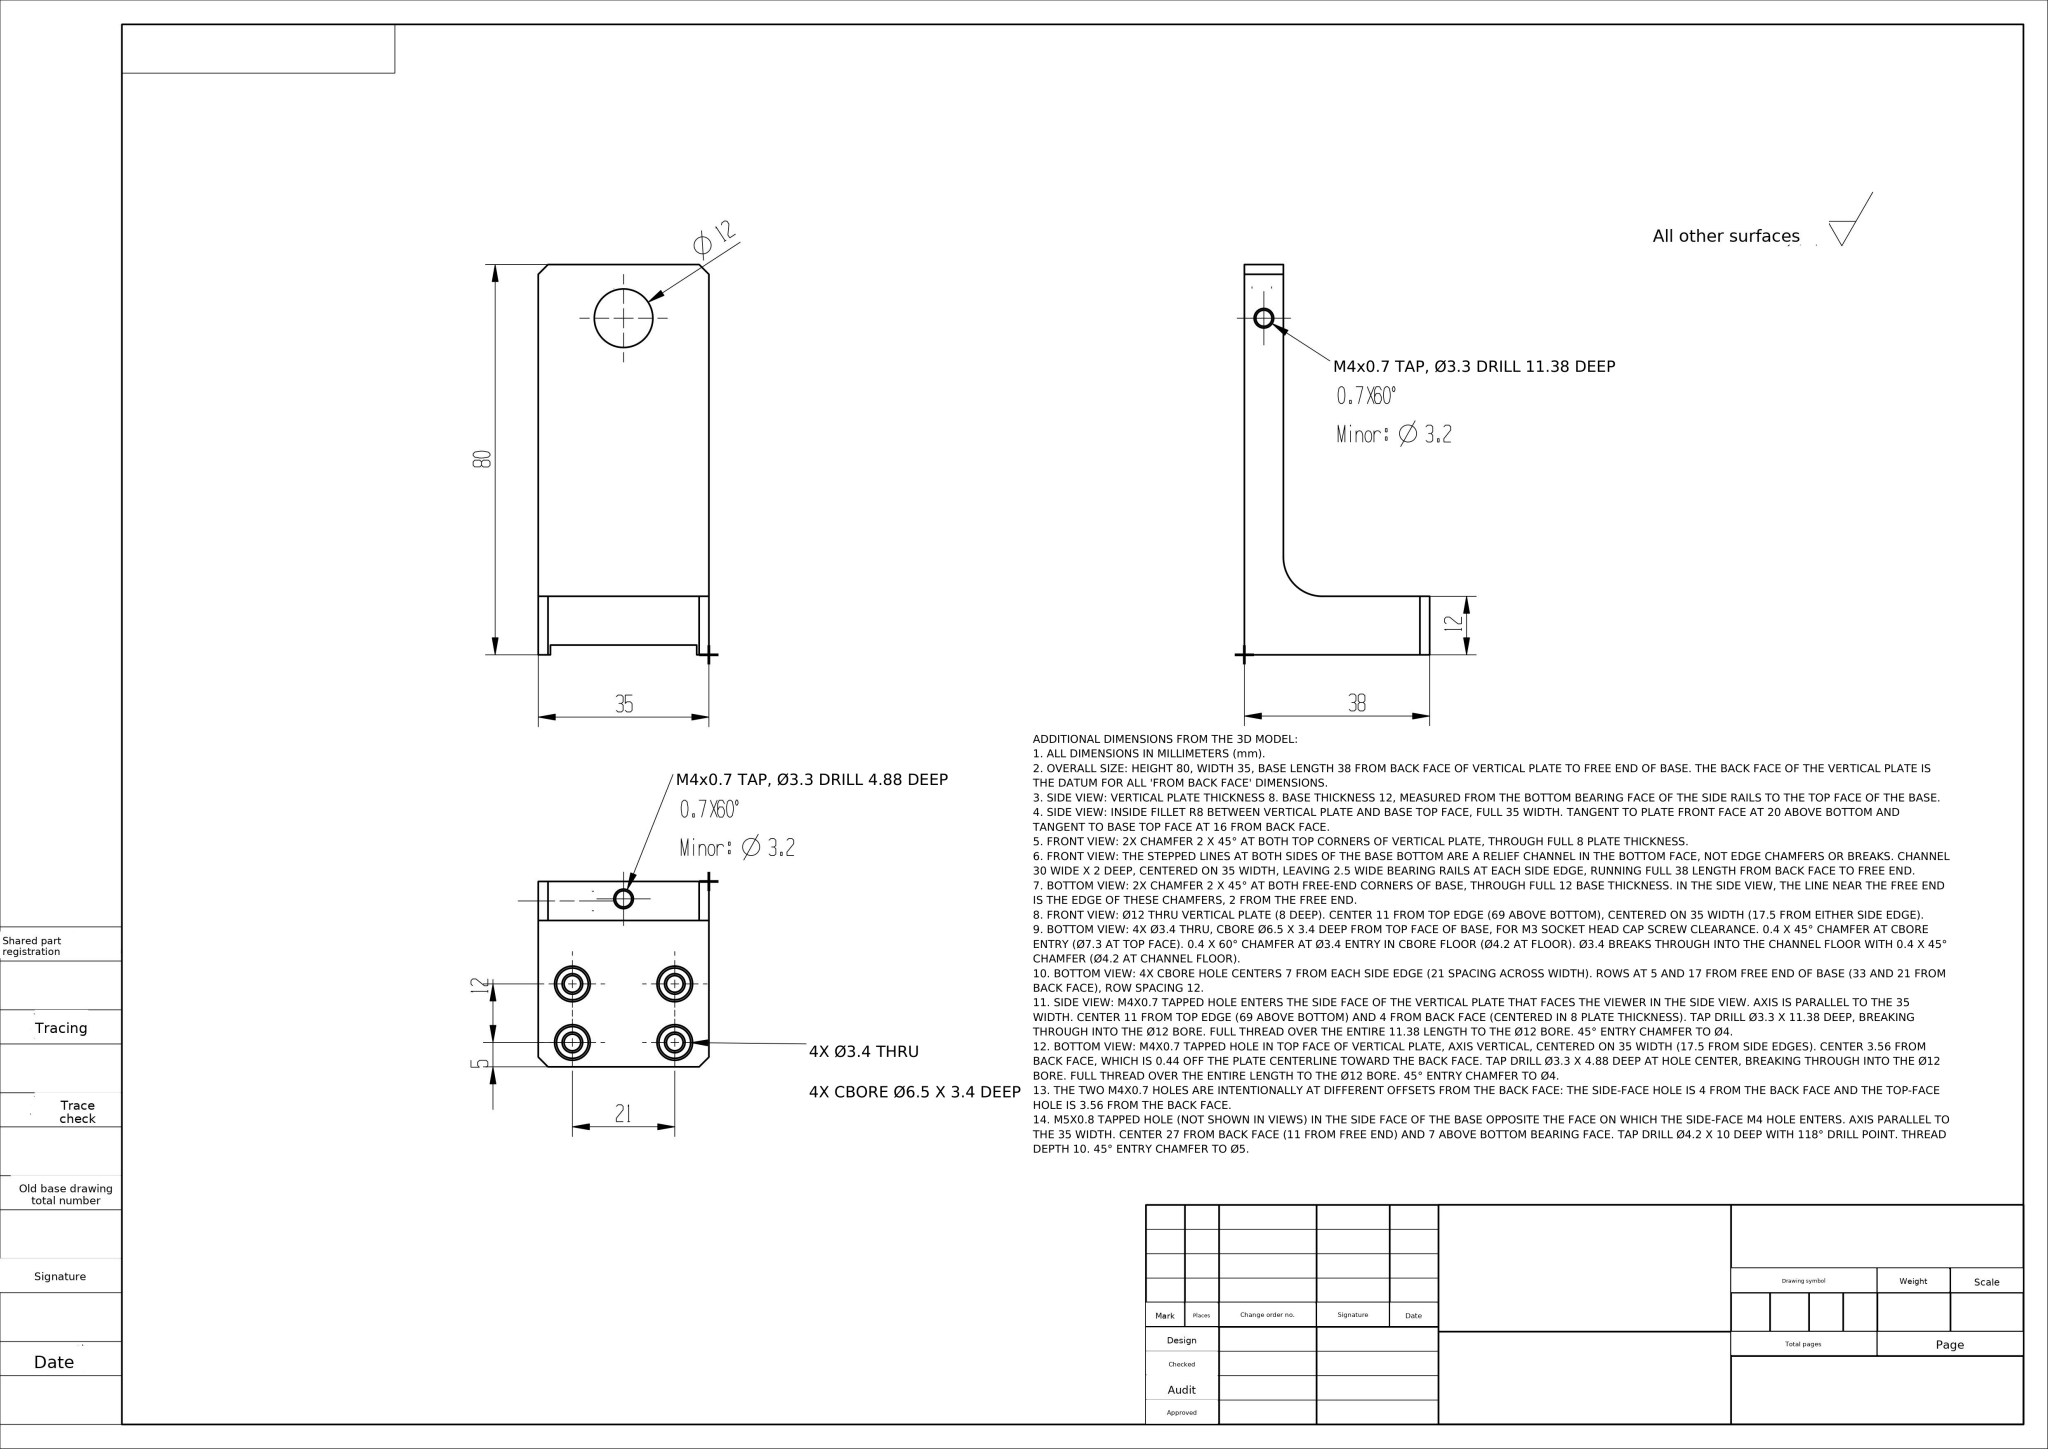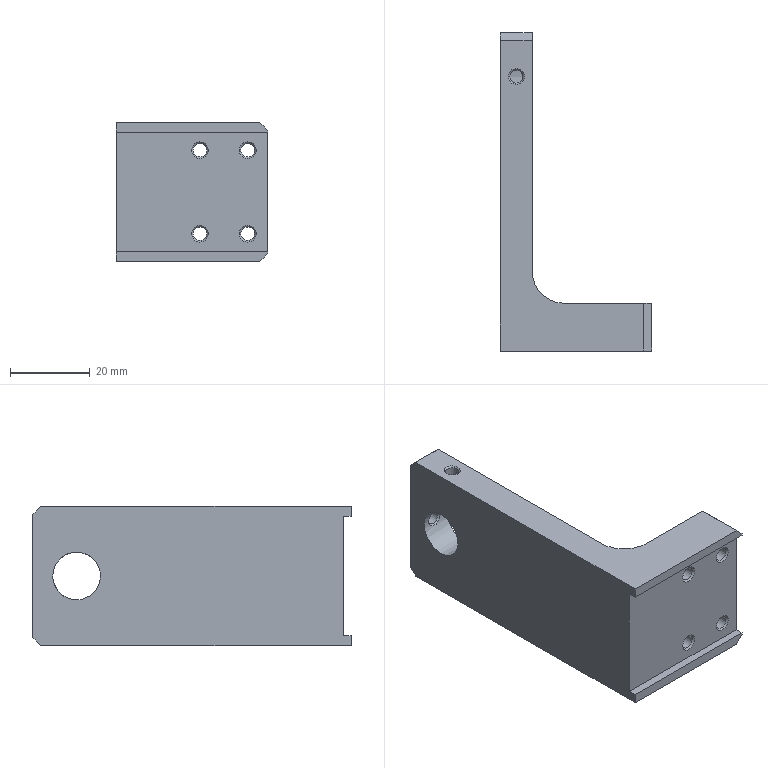Part | NX | mm | 1 solid | 51 faces | box 38 x 80 x 35 mm | volume 31218 mm3 | plane 20 | cone 16 | cylinder 13 | spline 2 | commonest cylinder face diameters 3.4 x4 6.5 x4 3.3 x2 16 x1 12 x1 4.2 x1